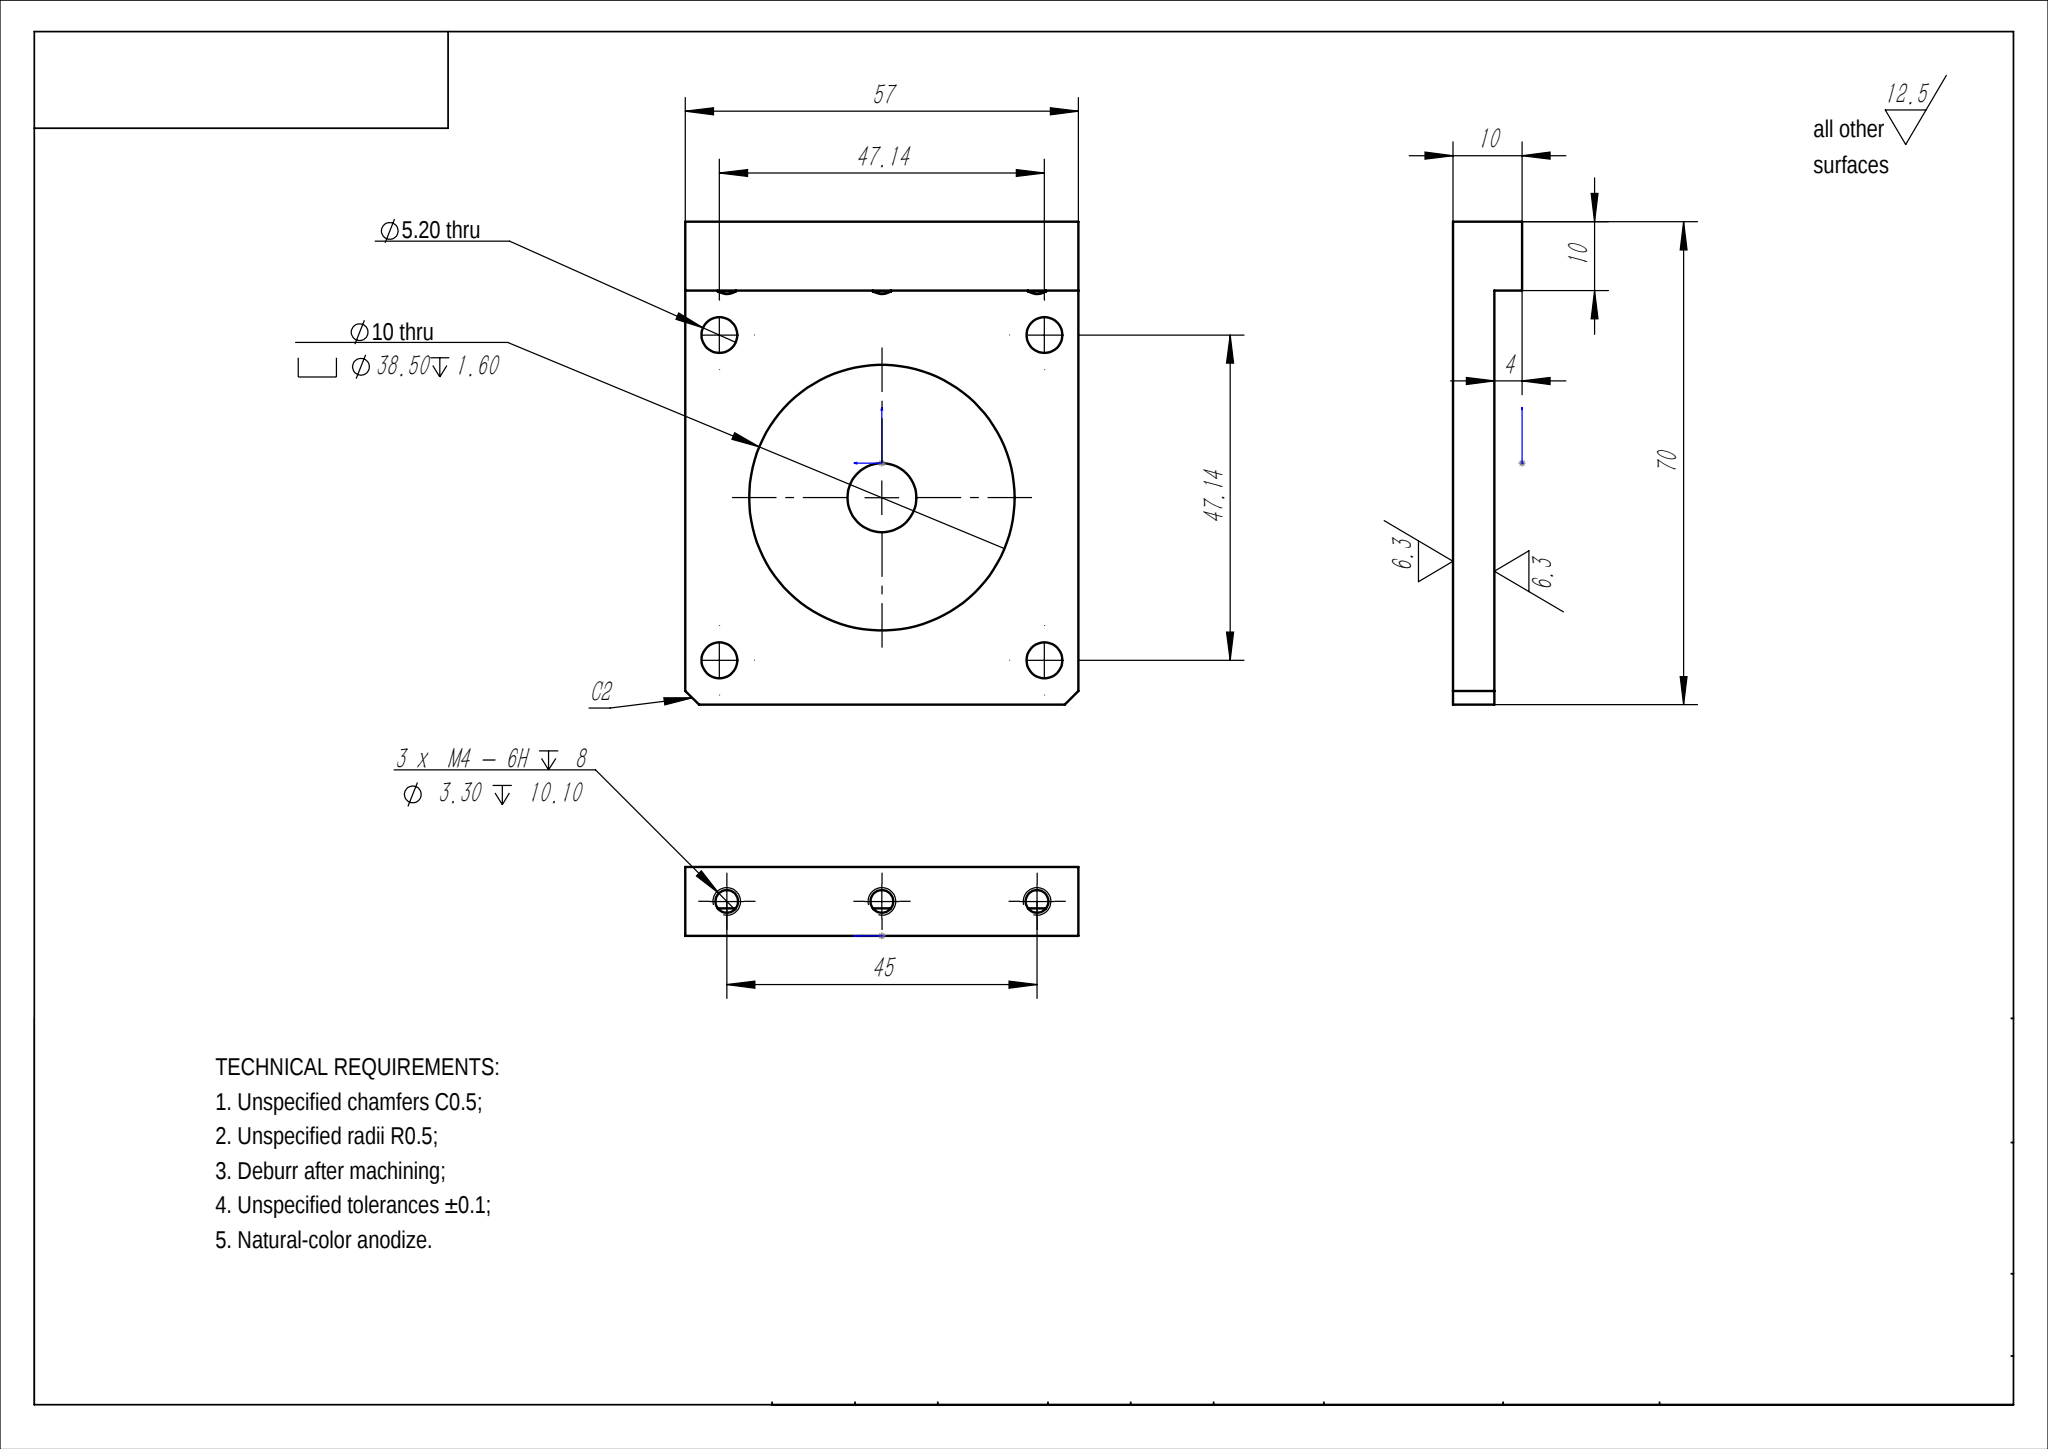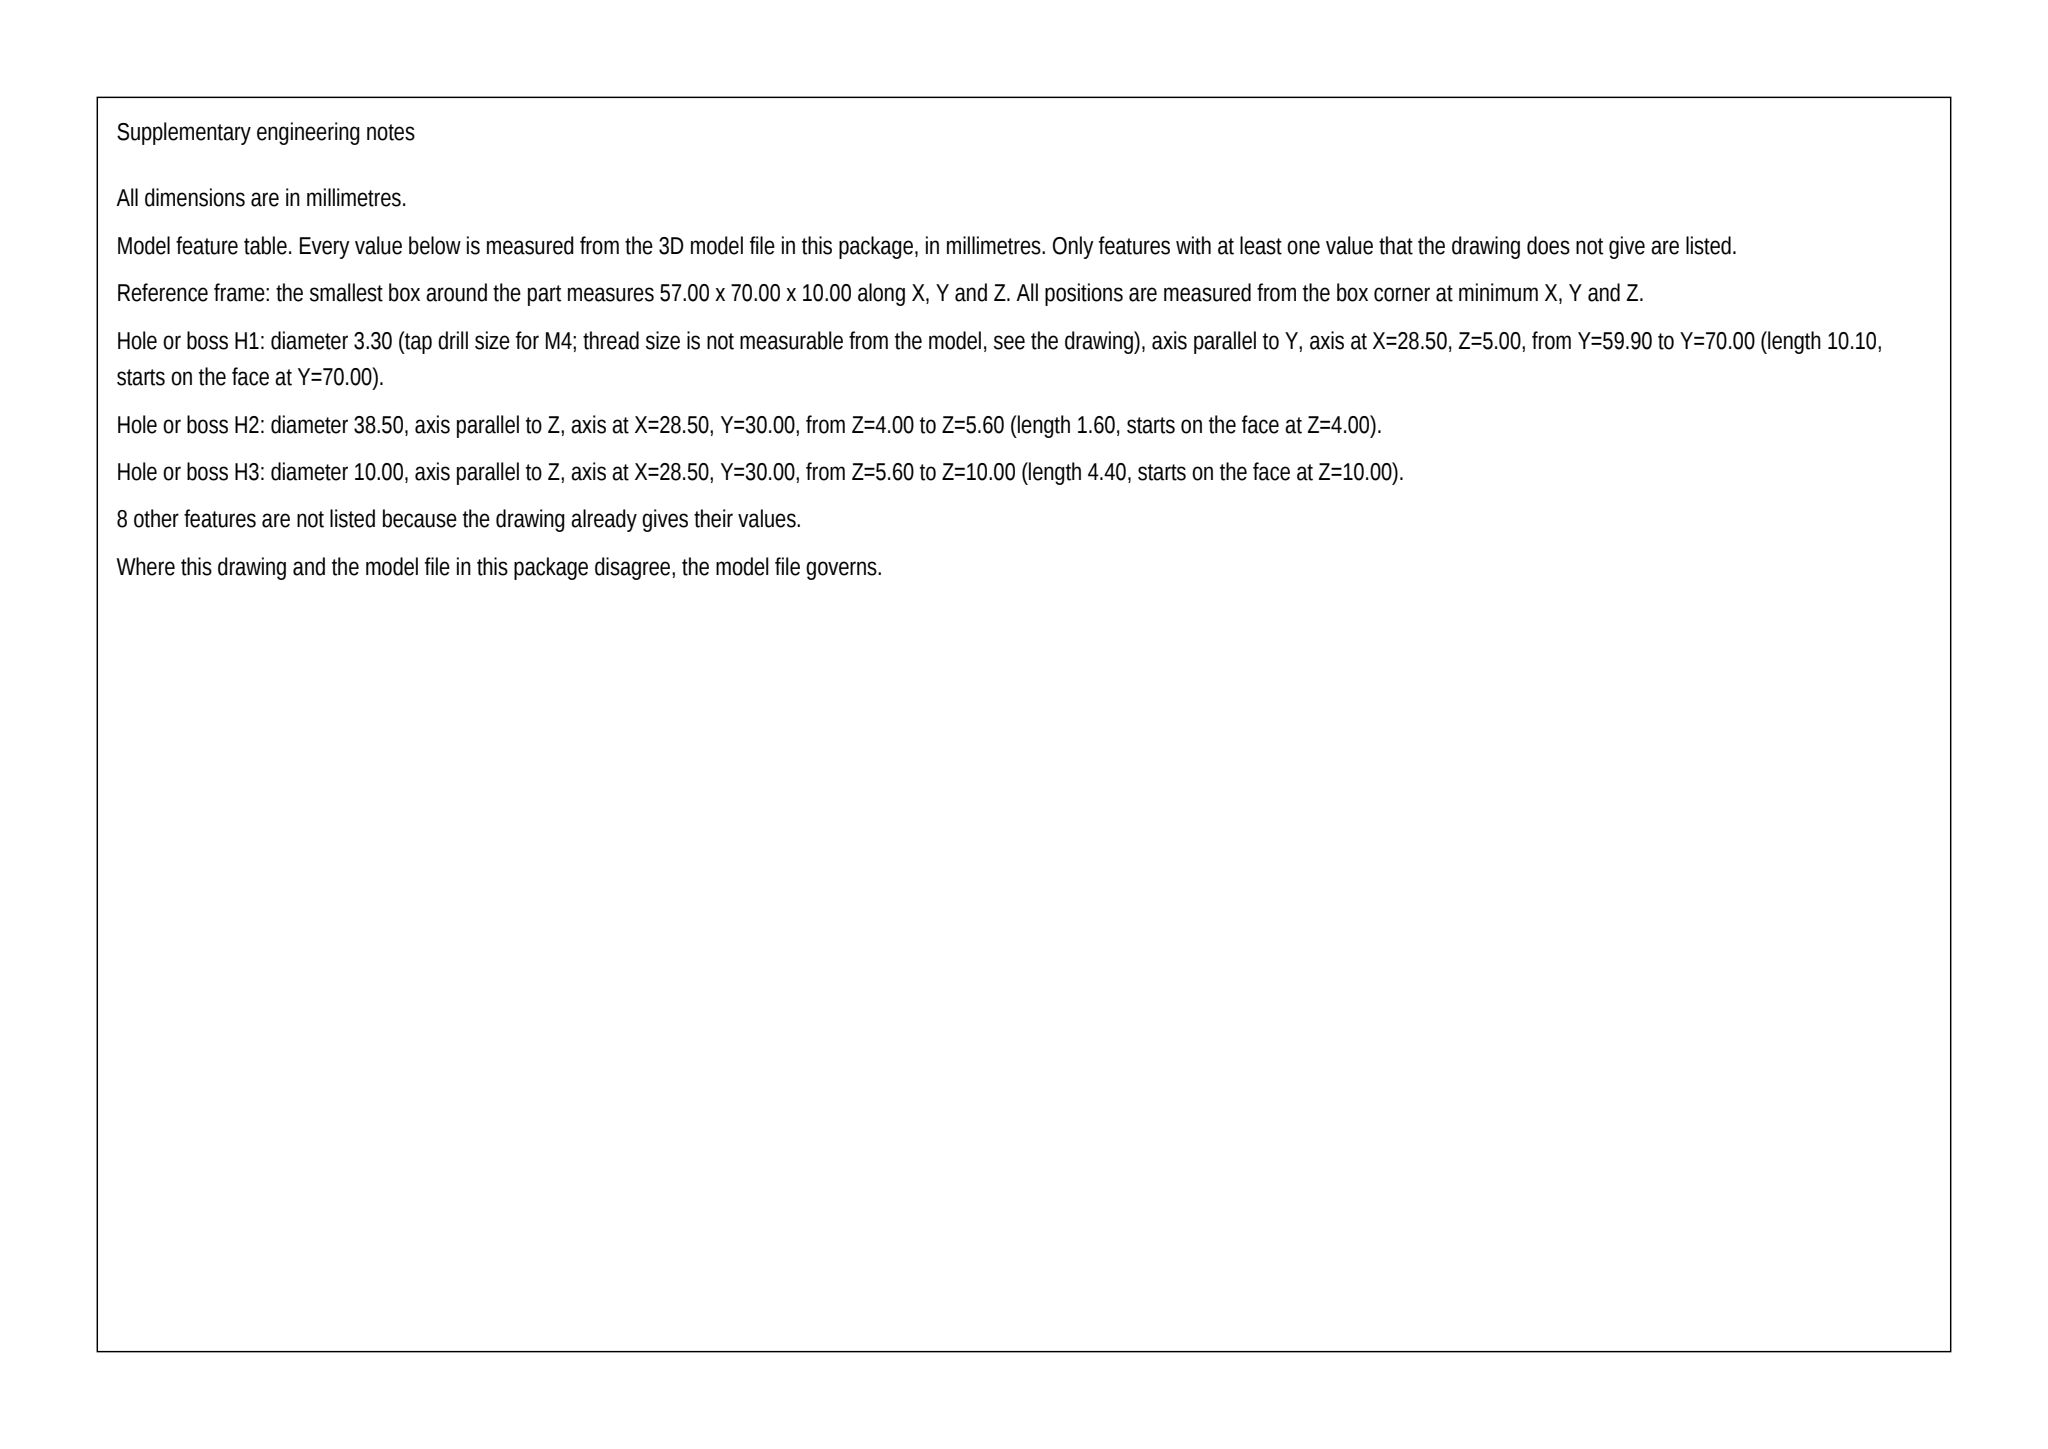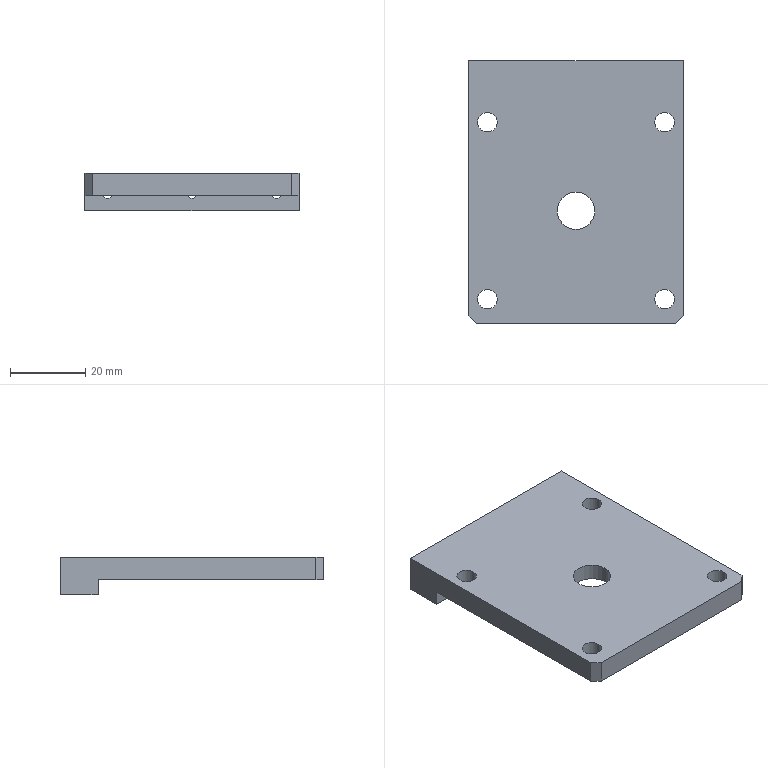Part | SolidWorks | mm | 1 solid | 35 faces | box 57 x 70 x 10 mm | volume 23211 mm3 | cylinder 18 | plane 11 | cone 6 | commonest cylinder face diameters 5.2 x8 3.3 x6 10 x2 38.5 x2
build123d program:
from build123d import *

# Parameters (mm, degrees)
SKETCH1_W             = 57
SKETCH1_H             = 70
BOSS_EXTRUDE1_DEPTH   = 10
M4_TAPPED_HOLE1_D     = 3.3
M4_TAPPED_HOLE1_DEPTH = 10.1
M4_TAPPED_HOLE1_TIP   = 0.9914
SKETCH4_R             = 19.25
CUT_EXTRUDE1_DEPTH    = 5.6
SKETCH5_R             = 5
CUT_EXTRUDE2_DEPTH    = 46.482
SKETCH6_R             = 2.6
CUT_EXTRUDE3_DEPTH    = 47.23
SKETCH7_W             = 57
SKETCH7_H             = 60
CUT_EXTRUDE4_DEPTH    = 4
CHAMFER1_SIZE         = 2


with BuildPart() as part:
    # Sketch1 → Boss-Extrude1 (new body)
    with BuildSketch(Plane.XY):
        Rectangle(SKETCH1_W, SKETCH1_H)
    extrude(amount=BOSS_EXTRUDE1_DEPTH)

    # M4 Tapped Hole1
    with Locations(Plane(origin=(0, 35, 0), x_dir=(1, 0, 0), z_dir=(0, 1, 0))):
        with Locations((-22.5, -5), (22.5, -5), (0, -5)):
            Hole(M4_TAPPED_HOLE1_D / 2, depth=M4_TAPPED_HOLE1_DEPTH)
            with Locations((0, 0, -(M4_TAPPED_HOLE1_DEPTH + M4_TAPPED_HOLE1_TIP / 2))):  # 118° drill point
                Cone(0, M4_TAPPED_HOLE1_D / 2, M4_TAPPED_HOLE1_TIP, mode=Mode.SUBTRACT)

    # Sketch4 → Cut-Extrude1 (cut)
    with BuildSketch(Plane.XY):
        with Locations((0, -5)):
            Circle(SKETCH4_R)
    extrude(amount=CUT_EXTRUDE1_DEPTH, mode=Mode.SUBTRACT)

    # Sketch5 → Cut-Extrude2 (cut, through all)
    with BuildSketch(Plane(origin=(0, 0, 5.6), x_dir=(-1, 0, 0), z_dir=(0, 0, -1))):
        with Locations((0, -5)):
            Circle(SKETCH5_R)
    extrude(amount=-CUT_EXTRUDE2_DEPTH, mode=Mode.SUBTRACT)

    # Sketch6 → Cut-Extrude3 (cut, through all)
    with BuildSketch(Plane.XY.offset(10)):
        with Locations((-23.57, 18.57)):
            Circle(SKETCH6_R)
        with Locations(Location((-23.57, -28.57, 0), (0, 0, 180))):
            Circle(SKETCH6_R)
        with Locations((23.57, -28.57)):
            Circle(SKETCH6_R)
        with Locations(Location((23.57, 18.57, 0), (0, 0, 180))):
            Circle(SKETCH6_R)
    extrude(amount=-CUT_EXTRUDE3_DEPTH, mode=Mode.SUBTRACT)

    # Sketch7 → Cut-Extrude4 (cut)
    with BuildSketch(Plane.XY):
        with Locations((0, -5)):
            Rectangle(SKETCH7_W, SKETCH7_H)
    extrude(amount=CUT_EXTRUDE4_DEPTH, mode=Mode.SUBTRACT)

    # Chamfer1
    chamfer1_edges = [part.edges().sort_by_distance(p)[0] for p in [
        (28.5, -35, 7),
        (-28.5, -35, 7),
    ]]
    chamfer(chamfer1_edges, length=CHAMFER1_SIZE)


solid = part.part